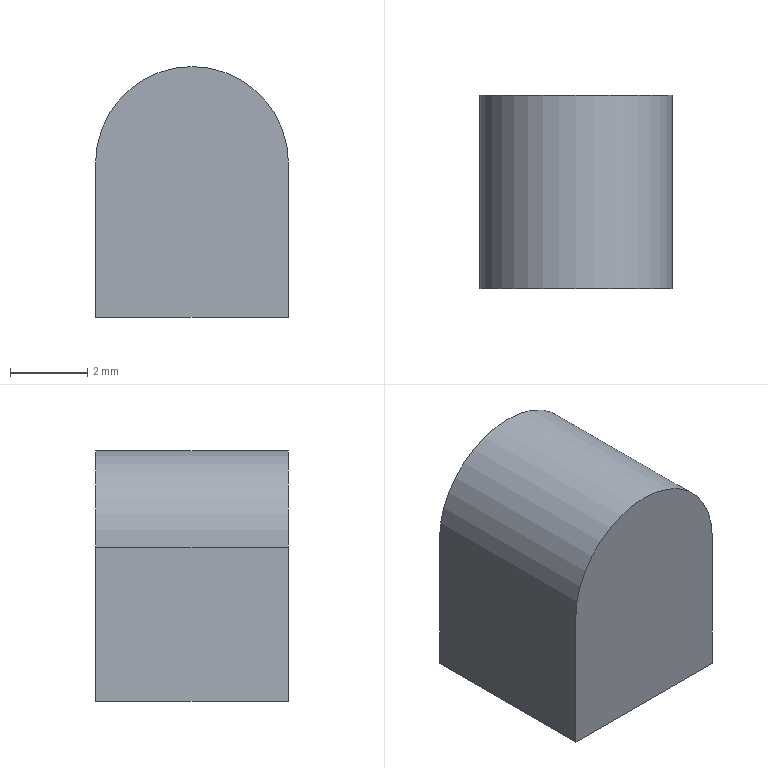Component | SolidWorks | MGL-PACK-03-00Fixture-1_MGL-PACK-03-04LimitBlock-1 | 1 solid | 6 faces | box 5 x 5 x 6.5 mm | volume 149 mm3 | plane 5 | cylinder 1 | commonest cylinder face diameters 5 x1
build123d program:
from build123d import *

# Parameters (mm, degrees)
BOSS_EXTRUDE1_DEPTH = 5


with BuildPart() as part:
    # Sketch1 → Boss-Extrude1 (new body)
    with BuildSketch(Plane.XY):
        with BuildLine():
            Line((-2.5, -2), (2.5, -2))
            Line((2.5, -2), (2.5, 2))
            ThreePointArc((2.5, 2), (0, 4.5), (-2.5, 2))
            Line((-2.5, 2), (-2.5, -2))
        make_face()
    extrude(amount=BOSS_EXTRUDE1_DEPTH)


solid = part.part

# Placed as in the assembly
solid = solid.moved(Location((225, 35, -263.3), (90, 0, 0)))
STEP:
#1=CARTESIAN_POINT('',(8.957,1.181,-10.287));
#2=VERTEX_POINT('',#1);
#3=CARTESIAN_POINT('',(8.957,1.181,-10.445));
#4=VERTEX_POINT('',#3);
#5=CARTESIAN_POINT('',(8.957,1.181,-10.445));
#6=DIRECTION('',(-0.,-0.,-1.));
#7=VECTOR('',#6,39.37);
#8=LINE('',#5,#7);
#9=EDGE_CURVE('',#2,#4,#8,.T.);
#10=ORIENTED_EDGE('',*,*,#9,.T.);
#11=CARTESIAN_POINT('',(8.957,1.378,-10.445));
#12=VERTEX_POINT('',#11);
#13=CARTESIAN_POINT('',(8.957,1.378,-10.445));
#14=DIRECTION('',(0.,-1.,0.));
#15=VECTOR('',#14,39.37);
#16=LINE('',#13,#15);
#17=EDGE_CURVE('',#12,#4,#16,.T.);
#18=ORIENTED_EDGE('',*,*,#17,.F.);
#19=CARTESIAN_POINT('',(8.957,1.378,-10.287));
#20=VERTEX_POINT('',#19);
#21=CARTESIAN_POINT('',(8.957,1.378,-10.445));
#22=DIRECTION('',(-0.,-0.,-1.));
#23=VECTOR('',#22,39.37);
#24=LINE('',#21,#23);
#25=EDGE_CURVE('',#20,#12,#24,.T.);
#26=ORIENTED_EDGE('',*,*,#25,.F.);
#27=CARTESIAN_POINT('',(8.957,1.378,-10.287));
#28=DIRECTION('',(0.,-1.,0.));
#29=VECTOR('',#28,39.37);
#30=LINE('',#27,#29);
#31=EDGE_CURVE('',#20,#2,#30,.T.);
#32=ORIENTED_EDGE('',*,*,#31,.T.);
#33=EDGE_LOOP('',(#10,#18,#26,#32));
#34=FACE_OUTER_BOUND('',#33,.T.);
#35=CARTESIAN_POINT('',(8.957,1.378,-10.445));
#36=DIRECTION('',(-1.,-0.,-0.));
#37=DIRECTION('',(0.,-1.,0.));
#38=AXIS2_PLACEMENT_3D('',#35,#36,#37);
#39=PLANE('',#38);
#40=ADVANCED_FACE('',(#34),#39,.F.);
#41=CARTESIAN_POINT('',(8.76,1.181,-10.445));
#42=VERTEX_POINT('',#41);
#43=CARTESIAN_POINT('',(8.957,1.181,-10.445));
#44=DIRECTION('',(-1.,-0.,-0.));
#45=VECTOR('',#44,39.37);
#46=LINE('',#43,#45);
#47=EDGE_CURVE('',#4,#42,#46,.T.);
#48=ORIENTED_EDGE('',*,*,#47,.T.);
#49=CARTESIAN_POINT('',(8.76,1.378,-10.445));
#50=VERTEX_POINT('',#49);
#51=CARTESIAN_POINT('',(8.76,1.378,-10.445));
#52=DIRECTION('',(0.,-1.,0.));
#53=VECTOR('',#52,39.37);
#54=LINE('',#51,#53);
#55=EDGE_CURVE('',#50,#42,#54,.T.);
#56=ORIENTED_EDGE('',*,*,#55,.F.);
#57=CARTESIAN_POINT('',(8.957,1.378,-10.445));
#58=DIRECTION('',(-1.,-0.,-0.));
#59=VECTOR('',#58,39.37);
#60=LINE('',#57,#59);
#61=EDGE_CURVE('',#12,#50,#60,.T.);
#62=ORIENTED_EDGE('',*,*,#61,.F.);
#63=ORIENTED_EDGE('',*,*,#17,.T.);
#64=EDGE_LOOP('',(#48,#56,#62,#63));
#65=FACE_OUTER_BOUND('',#64,.T.);
#66=CARTESIAN_POINT('',(8.957,1.378,-10.445));
#67=DIRECTION('',(0.,0.,1.));
#68=DIRECTION('',(-0.,1.,-0.));
#69=AXIS2_PLACEMENT_3D('',#66,#67,#68);
#70=PLANE('',#69);
#71=ADVANCED_FACE('',(#65),#70,.F.);
#72=CARTESIAN_POINT('',(8.76,1.181,-10.287));
#73=VERTEX_POINT('',#72);
#74=CARTESIAN_POINT('',(8.76,1.181,-10.445));
#75=DIRECTION('',(0.,0.,1.));
#76=VECTOR('',#75,39.37);
#77=LINE('',#74,#76);
#78=EDGE_CURVE('',#42,#73,#77,.T.);
#79=ORIENTED_EDGE('',*,*,#78,.T.);
#80=CARTESIAN_POINT('',(8.76,1.378,-10.287));
#81=VERTEX_POINT('',#80);
#82=CARTESIAN_POINT('',(8.76,1.378,-10.287));
#83=DIRECTION('',(0.,-1.,0.));
#84=VECTOR('',#83,39.37);
#85=LINE('',#82,#84);
#86=EDGE_CURVE('',#81,#73,#85,.T.);
#87=ORIENTED_EDGE('',*,*,#86,.F.);
#88=CARTESIAN_POINT('',(8.76,1.378,-10.445));
#89=DIRECTION('',(0.,0.,1.));
#90=VECTOR('',#89,39.37);
#91=LINE('',#88,#90);
#92=EDGE_CURVE('',#50,#81,#91,.T.);
#93=ORIENTED_EDGE('',*,*,#92,.F.);
#94=ORIENTED_EDGE('',*,*,#55,.T.);
#95=EDGE_LOOP('',(#79,#87,#93,#94));
#96=FACE_OUTER_BOUND('',#95,.T.);
#97=CARTESIAN_POINT('',(8.76,1.378,-10.445));
#98=DIRECTION('',(1.,0.,0.));
#99=DIRECTION('',(-0.,1.,-0.));
#100=AXIS2_PLACEMENT_3D('',#97,#98,#99);
#101=PLANE('',#100);
#102=ADVANCED_FACE('',(#96),#101,.F.);
#103=CARTESIAN_POINT('',(8.858,1.181,-10.287));
#104=DIRECTION('',(-0.,1.,-0.));
#105=DIRECTION('',(1.,0.,0.));
#106=AXIS2_PLACEMENT_3D('',#103,#104,#105);
#107=CIRCLE('',#106,0.09843);
#108=EDGE_CURVE('',#73,#2,#107,.T.);
#109=ORIENTED_EDGE('',*,*,#108,.T.);
#110=ORIENTED_EDGE('',*,*,#31,.F.);
#111=CARTESIAN_POINT('',(8.858,1.378,-10.287));
#112=DIRECTION('',(-0.,1.,-0.));
#113=DIRECTION('',(1.,0.,0.));
#114=AXIS2_PLACEMENT_3D('',#111,#112,#113);
#115=CIRCLE('',#114,0.09843);
#116=EDGE_CURVE('',#81,#20,#115,.T.);
#117=ORIENTED_EDGE('',*,*,#116,.F.);
#118=ORIENTED_EDGE('',*,*,#86,.T.);
#119=EDGE_LOOP('',(#109,#110,#117,#118));
#120=FACE_OUTER_BOUND('',#119,.T.);
#121=CARTESIAN_POINT('',(8.858,1.378,-10.287));
#122=DIRECTION('',(0.,-1.,0.));
#123=DIRECTION('',(1.,0.,0.));
#124=AXIS2_PLACEMENT_3D('',#121,#122,#123);
#125=CYLINDRICAL_SURFACE('',#124,0.09843);
#126=ADVANCED_FACE('',(#120),#125,.T.);
#127=ORIENTED_EDGE('',*,*,#25,.T.);
#128=ORIENTED_EDGE('',*,*,#61,.T.);
#129=ORIENTED_EDGE('',*,*,#92,.T.);
#130=ORIENTED_EDGE('',*,*,#116,.T.);
#131=EDGE_LOOP('',(#127,#128,#129,#130));
#132=FACE_OUTER_BOUND('',#131,.T.);
#133=CARTESIAN_POINT('',(8.858,1.378,-10.287));
#134=DIRECTION('',(0.,-1.,0.));
#135=DIRECTION('',(1.,0.,0.));
#136=AXIS2_PLACEMENT_3D('',#133,#134,#135);
#137=PLANE('',#136);
#138=ADVANCED_FACE('',(#132),#137,.F.);
#139=ORIENTED_EDGE('',*,*,#9,.F.);
#140=ORIENTED_EDGE('',*,*,#108,.F.);
#141=ORIENTED_EDGE('',*,*,#78,.F.);
#142=ORIENTED_EDGE('',*,*,#47,.F.);
#143=EDGE_LOOP('',(#139,#140,#141,#142));
#144=FACE_OUTER_BOUND('',#143,.T.);
#145=CARTESIAN_POINT('',(8.858,1.181,-10.287));
#146=DIRECTION('',(0.,-1.,0.));
#147=DIRECTION('',(1.,0.,0.));
#148=AXIS2_PLACEMENT_3D('',#145,#146,#147);
#149=PLANE('',#148);
#150=ADVANCED_FACE('',(#144),#149,.T.);
#151=CLOSED_SHELL('',(#40,#71,#102,#126,#138,#150));
#152=MANIFOLD_SOLID_BREP('',#151);
#153=CARTESIAN_POINT('',(0.,0.,0.));
#154=DIRECTION('',(0.,0.,1.));
#155=DIRECTION('',(1.,0.,0.));
#156=AXIS2_PLACEMENT_3D('',#153,#154,#155);
#157=(LENGTH_UNIT()NAMED_UNIT(*)SI_UNIT($,.METRE.));
#158=LENGTH_MEASURE_WITH_UNIT(LENGTH_MEASURE(0.0254),#157);
#159=DIMENSIONAL_EXPONENTS(1.,0.,0.,0.,0.,0.,0.);
#160=(CONVERSION_BASED_UNIT('',#158)LENGTH_UNIT()NAMED_UNIT(#159));
#161=UNCERTAINTY_MEASURE_WITH_UNIT(LENGTH_MEASURE(0.00001),#160,'','');
#162=(NAMED_UNIT(*)PLANE_ANGLE_UNIT()SI_UNIT($,.RADIAN.));
#163=(NAMED_UNIT(*)SI_UNIT($,.STERADIAN.)SOLID_ANGLE_UNIT());
#164=(GEOMETRIC_REPRESENTATION_CONTEXT(3)GLOBAL_UNCERTAINTY_ASSIGNED_CONTEXT((#161))GLOBAL_UNIT_ASSIGNED_CONTEXT((#160,#162,#163))REPRESENTATION_CONTEXT('',''));
#165=ADVANCED_BREP_SHAPE_REPRESENTATION('',(#152,#156),#164);
#166=COLOUR_RGB('',0.7922,0.8196,0.9333);
#167=FILL_AREA_STYLE_COLOUR('',#166);
#168=FILL_AREA_STYLE('',(#167));
#169=SURFACE_STYLE_FILL_AREA(#168);
#170=SURFACE_SIDE_STYLE('',(#169));
#171=SURFACE_STYLE_USAGE(.BOTH.,#170);
#172=PRESENTATION_STYLE_ASSIGNMENT((#171));
#173=STYLED_ITEM('',(#172),#152);
#174=PRESENTATION_LAYER_ASSIGNMENT('','',(#173));
#175=(LENGTH_UNIT()NAMED_UNIT(*)SI_UNIT($,.METRE.));
#176=LENGTH_MEASURE_WITH_UNIT(LENGTH_MEASURE(0.0254),#175);
#177=DIMENSIONAL_EXPONENTS(1.,0.,0.,0.,0.,0.,0.);
#178=(CONVERSION_BASED_UNIT('',#176)LENGTH_UNIT()NAMED_UNIT(#177));
#179=UNCERTAINTY_MEASURE_WITH_UNIT(LENGTH_MEASURE(0.00001),#178,'','');
#180=(NAMED_UNIT(*)PLANE_ANGLE_UNIT()SI_UNIT($,.RADIAN.));
#181=(NAMED_UNIT(*)SI_UNIT($,.STERADIAN.)SOLID_ANGLE_UNIT());
#182=(GEOMETRIC_REPRESENTATION_CONTEXT(3)GLOBAL_UNCERTAINTY_ASSIGNED_CONTEXT((#179))GLOBAL_UNIT_ASSIGNED_CONTEXT((#178,#180,#181))REPRESENTATION_CONTEXT('',''));
#183=MECHANICAL_DESIGN_GEOMETRIC_PRESENTATION_REPRESENTATION('',(#173),#182);